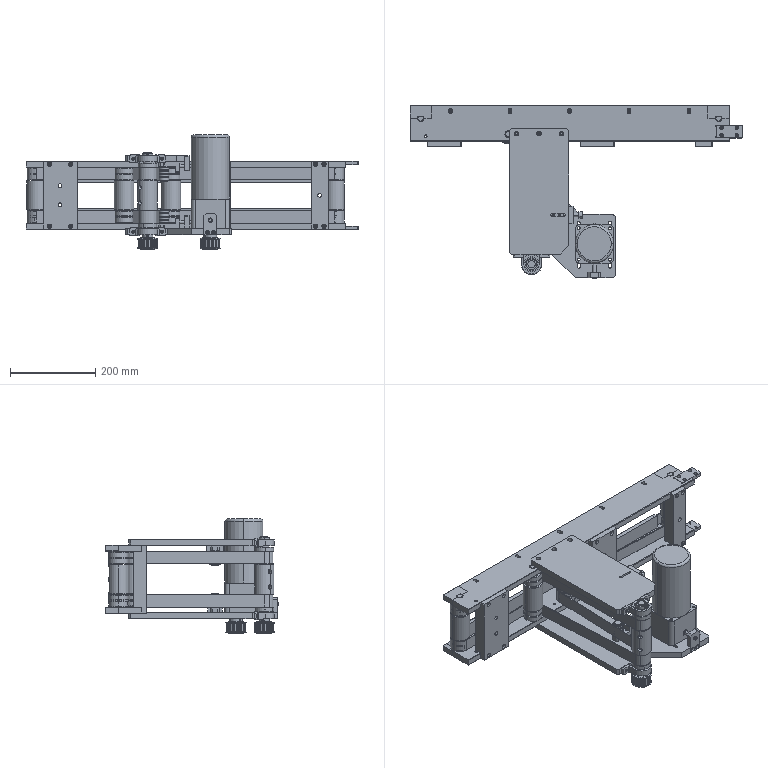Assembly | SolidWorks | mm | 105 component files | 105 solids | 2713 faces | box 780 x 408 x 268 mm | volume 7374676 mm3 | cylinder 1325 | plane 933 | cone 249 | torus 206 | commonest cylinder face diameters 15 x136 3.3 x76 1.06 x74 1.72 x73 8 x70 37.9 x64 19.7 x64 4.2 x60
Bill of materials:
ATPA15L075_A_H15-01-2 | 1 |  | Toothed pulley-like body: cylindrical hub with axial teeth/grooves around its outside, a flange at each end with an angled (chamfered) rim, and a central bore with one keyway. No extended hub.
ATPA15L075_B_H15-2 | 1 |  | Toothed pulley-like body with flanges at both ends and an extended cylindrical hub on one side. Has a central keyed bore and a radial hole through the hub.
Belt4-15^SW-111 | 1 |  | Thin-walled closed-loop band shaped like a T in plan, with a long crossbar and a tapering stem, all ends rounded; open in the middle (outline-wall only, no floor visible).
Belt5-16^SW-111 | 1 |  | Thin-walled closed-loop band shaped like a T in plan, with a long crossbar and a tapering stem, rounded ends; hollow interior.
hex head bolts-full thread grade c gb | 1 |  | Hex-head bolt-like part: hexagonal head with chamfered top corners and a round bearing face underneath, plus a plain cylindrical shank with a chamfered tip.
JBM5120-502-01-2 | 1 |  | Tall cylindrical body with a rounded top edge, sitting on a square block/flange with rounded corners and four corner through-holes; a small stepped boss and a thin round shaft stick out of the bottom face.
M8Screw-2 | 2 |  | Headed pin: a plain cylindrical shank ending in a shorter, larger-diameter cylindrical head with a flat end face.
Headless_pin_DIN_913_M4x4-2 | 4 |  | Short solid cylinder with a hexagonal socket recess in one end; both ends are chamfered, one more heavily (conical) than the other.
PBT17x-2 | 2 |  | Housing with a cylindrical body and a central through-bore, plus two side mounting ears that each have a through-hole; a round boss sticks out from one face, and the ears sit on a raised base line.
B6302ZZ-2 | 16 |  | Annular ring/disc with a central bore and rounded outer edges; the face has a raised inner rim and outer rim with a shallow recessed annulus between them.
XT-1-08-2 | 2 |  | Long slender cylindrical pin with chamfered ends and a small radial cross-hole near mid-length.
XT-1-09-2 | 24 |  | Thin flat ring (washer-like annulus) with rectangular cross-section and no visible chamfers.
XT-1-11-2 | 2 |  | Cylindrical sleeve/spacer with a coaxial through-bore and small chamfers on the outer end edges.
XT-1-07-2 | 2 |  | Long slender cylindrical pin with a small radial cross-hole near mid-length and a flat (D-cut) running along part of its length; ends chamfered.
XT-1-10-2 | 2 |  | Plain cylindrical sleeve/spacer with a concentric through bore and small chamfers on both outer end edges.
B6901ZZ-2 | 8 |  | Short thick ring with a concentric bore and a thin circular groove on the end face, between the bore and the outer edge. Slightly faceted mesh surface.
XT-1-20-2 | 2 |  | Rectangular block with a stepped, L-shaped side profile: a long thinner arm with one rounded end, and a taller square section at the other end. The arm has an elongated through opening with flat sides, a round through hole, and a cross hole in its side face.
XT-1-21-2 | 2 |  | Headed cylindrical pin: a short larger-diameter disc head on a long round shank, with a flat cut on one side of the shank near the end opposite the head.
XT-1-22-2 | 8 |  | Thin flat annular ring/washer with a large central opening and square-cut edges.
XT-1-01-2 | 1 |  | Long, narrow rectangular bar/plate with stepped notched ends, a row of oblong slots, several round holes of various sizes, small holes in the side edge, and a rectangular pocket/recess at one end.
XT-1-02-2 | 1 |  | Long, narrow rectangular bar/plate almost the same as the companion bar: stepped notched ends, a row of small slots, round holes near the middle and small side holes. The end recess looks oriented on the opposite side.
XT-1-03-2 | 2 |  | Rectangular plate with a rebated (stepped) back: a raised rectangular boss or land runs across the middle of one face. Has six through holes: four small ones near the corners and two larger ones on the centreline.
XT-1-04-2 | 1 |  | Long, slender strip with an L-shaped (angle) cross-section that has a small lip at the top. Ends have small chamfers. No holes are visible.
XT-1-05-2 | 1 |  | Long, slender strip with an L-shaped cross-section: a tall web and a short foot. A row of small, evenly spaced holes runs along its top edge.
XT-1-06-2 | 1 |  | Elongated rectangular bar or block with a stepped profile: a thinner full-length plate section carries a thicker raised section that stops short of both ends. The ends form thin flange steps. The flat face has four small through holes, one near each corner, and one larger hole in the middle.
XT-1-12-2 | 1 |  | Flat plate of even thickness with an irregular outline. A rectangular main area joins, through an angled (chamfered) edge transition, an offset rectangular extension. The extension has a large obround (slot-shaped) central cutout with four parallel elongated slots around it. The plate also has an extra slot, small holes, a rectangular notch in one edge, broken corners and small holes drilled into the edges.
XT-1-13-2 | 1 |  | Long, slender solid cylindrical shaft. One end steps down to a shorter section with a smaller diameter. Several small radial holes or dimples sit along the main length.
XT-1-14-2 | 1 |  | Stepped cylindrical sleeve with an axial bore through it. A wider band sits in the middle, with smaller-diameter ends on both sides. Three small axial holes are spaced around the end face, and the middle band has radial holes.
XT-1-15-2 | 2 |  | Round flanged disc. A smaller cylindrical boss projects from one face, a central bore runs through the part, and three holes pass through the flange.
XT-1-16-2 | 1 |  | Elongated prismatic bar or key-like block. One end is rounded into a half-round profile, and the other end looks flat or slightly angled.
XT-1-17-2 | 1 |  | Thick rectangular block. Two corners at one end are chamfered. A larger hole passes through near the chamfered end, and two smaller holes pass through near the opposite end.
XT-1-18-2 | 4 |  | Rectangular block with a semicircular U-shaped notch cut through one long edge. Two cross holes run through the block on either side of the notch, and the edges are bevelled or chamfered.
XT-1-19-2 | 1 |  | Rectangular plate or block with chamfered corners and one central through hole.
XT-1-23-2 | 1 |  | Rectangular plate or block with chamfered corners. Two smaller through holes sit near one edge, and one larger hole sits centred near the opposite edge.
XT-1-24-2 | 2 |  | Flat rectangular plate with four chamfered corners and four through holes in a rectangular pattern.
XT-1-25-2 | 1 |  | Thin, elongated rectangular plate. It has corner chamfers, one of them larger, a row of three holes along one short edge and an elongated slot near one long edge. Small holes are drilled into the side edges, and a shallow step or rebate runs along part of one edge.
Mates:
1. coincident | XT-1-01-2-1 face at (214.283, 139.385, 7.5) dir (-1, 0, 0) | XT-1-02-2-1 face at (214.283, 139.385, -138) dir (-1, 0, 0)
2. coincident | XT-1-01-2-1 face at (214.283, 54.385, 7.5) dir (0, -1, 0) | XT-1-02-2-1 face at (214.283, 54.385, -138) dir (0, -1, 0)
3. distance | XT-1-02-2-1 face at (214.283, 139.385, -138) dir (0, 0, 1) | XT-1-01-2-1 face at (214.283, 139.385, -7.5) dir (0, 0, -1)
4. coincident | XT-1-01-2-1 face at (214.283, 54.385, 7.5) dir (0, -1, 0) | XT-1-03-2-1 face at (334.283, 54.385, 7.5) dir (0, 1, 0)
5. coincident | XT-1-02-2-1 face at (214.283, 139.385, -138) dir (0, 0, 1) | XT-1-04-2-1 face at (909.283, 121.385, -138) dir (0, 0, -1)
6. distance | XT-1-04-2-1 face at (909.283, 129.385, -138) dir (0, 1, 0) | XT-1-02-2-1 face at (214.283, 139.385, -138) dir (0, 1, 0)
7. width | XT-1-04-2-1 face at (909.283, 131.385, -103) dir (1, 0, 0) | XT-1-04-2-1 face at (269.283, 131.385, -103) dir (-1, 0, 0) | XT-1-02-2-1 face at (214.283, 139.385, -138) dir (-1, 0, 0) | XT-1-02-2-1 face at (964.283, 139.385, -138) dir (1, 0, 0)
8. coincident | XT-1-01-2-1 face at (214.283, 139.385, -7.5) dir (0, 0, -1) | XT-1-05-2-1 face at (269.283, 121.385, -7.5) dir (0, 0, 1)
9. distance | XT-1-05-2-1 face at (269.283, 129.385, -7.5) dir (0, 1, 0) | XT-1-01-2-1 face at (214.283, 139.385, 7.5) dir (0, 1, 0)
10. width | XT-1-05-2-1 face at (909.283, 131.385, -42.5) dir (1, 0, 0) | XT-1-05-2-1 face at (269.283, 131.385, -42.5) dir (-1, 0, 0) | XT-1-01-2-1 face at (964.283, 139.385, 7.5) dir (1, 0, 0) | XT-1-01-2-1 face at (214.283, 139.385, 7.5) dir (-1, 0, 0)
11. coincident | XT-1-01-2-1 face at (214.283, 54.385, 7.5) dir (0, -1, 0) | XT-1-06-2-1 face at (924.283, 54.385, -138) dir (0, 1, 0)
12. concentric | XT-1-01-2-1 face at (239.283, 108.385, -7.5) dir (0, 0, 1) r 7.5 | Roller-2-1/XT-1-07-2-1 face at (239.283, 108.385, 7.5) dir (0, 0, -1) r 7.5
13. coincident | XT-1-01-2-1 face at (214.283, 139.385, 7.5) dir (0, 0, 1) | Roller-2-1/XT-1-07-2-1 face at (239.283, 108.385, 7.5) dir (0, 0, 1)
14. parallel | XT-1-01-2-1 face at (214.283, 108.385, -7.5) dir (0, 1, 0) | Roller-2-1/XT-1-07-2-1 face at (233.693, 113.385, -7.5) dir (0, 1, 0)
15. concentric | XT-1-01-2-1 face at (939.283, 108.385, -7.5) dir (0, 0, 1) r 7.5 | Roller-2-2/XT-1-07-2-1 face at (939.283, 108.385, 7.5) dir (0, 0, -1) r 7.5
16. coincident | XT-1-01-2-1 face at (214.283, 139.385, 7.5) dir (0, 0, 1) | Roller-2-2/XT-1-07-2-1 face at (939.283, 108.385, 7.5) dir (0, 0, 1)
17. parallel | XT-1-01-2-1 face at (964.283, 108.385, -7.5) dir (0, 1, 0) | Roller-2-2/XT-1-07-2-1 face at (933.693, 113.385, -7.5) dir (0, 1, 0)
18. concentric | XT-1-01-2-1 face at (444.783, 71.385, -7.5) dir (0, 0, 1) r 7.5 | Roller-01-2-1/XT-1-08-2-1 face at (444.783, 71.385, 7.5) dir (0, 0, -1) r 7.5
19. coincident | XT-1-01-2-1 face at (214.283, 139.385, 7.5) dir (0, 0, 1) | Roller-01-2-1/XT-1-08-2-1 face at (444.783, 71.385, 7.5) dir (0, 0, 1)
20. concentric | XT-1-01-2-1 face at (554.783, 71.385, -7.5) dir (0, 0, 1) r 7.5 | Roller-01-2-2/XT-1-08-2-1 face at (554.783, 71.385, 7.5) dir (0, 0, -1) r 7.5
21. coincident | XT-1-01-2-1 face at (214.283, 139.385, 7.5) dir (0, 0, 1) | Roller-01-2-2/XT-1-08-2-1 face at (554.783, 71.385, 7.5) dir (0, 0, 1)
22. coincident | XT-1-02-2-1 face at (214.283, 139.385, -153) dir (0, 0, -1) | XT-1-12-2-1 face at (447.283, 54.385, -153) dir (0, 0, 1)
23. concentric | XT-1-02-2-1 face at (464.283, 72.385, -153) dir (0, 0, -1) r 2.5 | XT-1-12-2-1 face at (464.283, 72.385, -166) dir (0, 0, -1) r 3.3
24. concentric | XT-1-02-2-1 face at (570.283, 72.385, -153) dir (0, 0, -1) r 2.5 | XT-1-12-2-1 face at (570.283, 72.385, -166) dir (0, 0, -1) r 3.3
25. coincident | XT-1-01-2-1 face at (214.283, 139.385, 7.5) dir (0, 0, 1) | XT-1-25-2-1 face at (587.283, 54.385, 7.5) dir (0, 0, -1)
26. concentric | XT-1-01-2-1 face at (570.283, 72.385, 7.5) dir (0, 0, 1) r 2.5 | XT-1-25-2-1 face at (570.283, 72.385, 20.5) dir (0, 0, 1) r 5.5
27. concentric | XT-1-01-2-1 face at (464.283, 72.385, 7.5) dir (0, 0, 1) r 2.5 | XT-1-25-2-1 face at (464.283, 72.385, 20.5) dir (0, 0, 1) r 5.5
28. coincident | XT-1-12-2-1 face at (547.283, -210.615, -151) dir (0, -1, 0) | PBT17-2-1/PBT17x-2-1 face at (457.283, -210.615, -167.5) dir (0, 1, 0)
29. concentric | XT-1-12-2-1 face at (533.283, -210.615, -158.5) dir (0, -1, 0) r 2.5 | PBT17-2-1/PBT17x-2-1 face at (533.283, -219.615, -158.5) dir (0, 1, 0) r 3.5
30. concentric | XT-1-12-2-1 face at (466.283, -210.615, -158.5) dir (0, -1, 0) r 2.5 | PBT17-2-1/PBT17x-2-1 face at (466.283, -219.615, -158.5) dir (0, 1, 0) r 3.5
31. coincident | XT-1-25-2-1 face at (447.283, -210.615, 20.5) dir (0, -1, 0) | PBT17-2-2/PBT17x-2-1 face at (542.283, -210.615, 22) dir (0, 1, 0)
32. concentric | XT-1-25-2-1 face at (466.283, -210.615, 13) dir (0, -1, 0) r 2.5 | PBT17-2-2/PBT17x-2-1 face at (466.283, -219.615, 13) dir (0, 1, 0) r 3.5
33. concentric | XT-1-25-2-1 face at (533.283, -210.615, 13) dir (0, -1, 0) r 2.5 | PBT17-2-2/PBT17x-2-1 face at (533.283, -219.615, 13) dir (0, 1, 0) r 3.5
34. concentric | PBT17-2-1/PBT17x-2-1 face at (499.783, -234.615, -153.5) dir (0, 0, -1) r 8.5 | XT-1-13-2-1 face at (499.783, -234.615, -199) dir (0, 0, -1) r 8.5
35. distance | XT-1-13-2-1 face at (499.783, -234.615, 28.5) dir (0, 0, 1) | PBT17-2-2/PBT17x-2-1 face at (499.783, -246.865, 25.5) dir (0, 0, 1)
36. concentric | XT-1-13-2-1 face at (499.783, -234.615, -199) dir (0, 0, -1) r 8.5 | XT-1-14-2-1 face at (499.783, -234.615, -138.5) dir (0, 0, 1) r 8.5
37. concentric | XT-1-13-2-1 face at (492.915, -239.623, -90.75) dir (-0.8081, -0.5891, 0) r 2.6 | XT-1-14-2-1 face at (481.602, -247.87, -90.75) dir (-0.8081, -0.5891, 0) r 2.75
38. concentric | XT-1-13-2-1 face at (499.783, -234.615, -199) dir (0, 0, -1) r 8.5 | XT-1-15-2-1 face at (499.783, -234.615, -138.5) dir (0, 0, -1) r 8.5
39. concentric | XT-1-14-2-1 face at (484.868, -236.208, -138.5) dir (0, 0, -1) r 1.65 | XT-1-15-2-1 face at (484.868, -236.208, -148.5) dir (0, 0, -1) r 4
40. coincident | XT-1-14-2-1 face at (488.001, -218.454, -138.5) dir (0, 0, -1) | XT-1-15-2-1 face at (499.783, -234.615, -138.5) dir (0, 0, 1)
41. concentric | XT-1-13-2-1 face at (499.783, -234.615, -199) dir (0, 0, -1) r 8.5 | XT-1-15-2-2 face at (499.783, -234.615, -7) dir (0, 0, 1) r 8.5
42. concentric | XT-1-14-2-1 face at (493.705, -248.328, -7) dir (0, 0, 1) r 1.65 | XT-1-15-2-2 face at (493.705, -248.328, 3) dir (0, 0, 1) r 4
43. coincident | XT-1-14-2-1 face at (499.783, -234.615, -7) dir (0, 0, 1) | XT-1-15-2-2 face at (499.783, -234.615, -7) dir (0, 0, -1)
44. coincident | XT-1-12-2-1 face at (447.283, 84.385, -151) dir (0, 0, 1) | JBM5120-502-01-2-1 face at (692.283, -231.615, -151) dir (0, 0, -1)
45. width | XT-1-12-2-1 face at (680.533, -136.615, -151) dir (1, 0, 0) | XT-1-12-2-1 face at (687.533, -136.615, -151) dir (-1, 0, 0) | JBM5120-502-01-2-1 face at (684.033, -149.865, 69) dir (0, 0, -1) r 3.5
46. width | XT-1-12-2-1 face at (607.033, -136.615, -151) dir (1, 0, 0) | XT-1-12-2-1 face at (614.033, -136.615, -151) dir (-1, 0, 0) | JBM5120-502-01-2-1 face at (610.533, -149.865, 69) dir (0, 0, -1) r 3.5
47. distance | JBM5120-502-01-2-1 face at (692.283, -141.615, -81.5) dir (0, 1, 0) | XT-1-12-2-1 face at (697.283, -116.615, -166) dir (0, 1, 0)
48. concentric | XT-1-13-2-1 face at (499.783, -234.615, -199) dir (0, 0, -1) r 7.5 | ATPA15L075_A_H15-01-2-1 face at (499.783, -234.615, -211) dir (0, 0, 1) r 7.5
49. coincident | XT-1-13-2-1 face at (504.202, -240.676, -199) dir (0, 0, -1) | ATPA15L075_A_H15-01-2-1 face at (494.776, -227.747, -199) dir (0, 0, -1)
50. coincident | XT-1-13-2-1 face at (497.132, -230.979, -199) dir (-0.5891, 0.8081, 0) | XT-1-16-2-1 face at (497.132, -230.979, -175) dir (0.5891, -0.8081, 0)
51. coincident | XT-1-13-2-1 face at (495.516, -232.157, -199) dir (0.8081, 0.5891, 0) | XT-1-16-2-1 face at (492.571, -228.117, -175) dir (-0.8081, -0.5891, 0)
52. coincident | XT-1-13-2-1 face at (504.202, -240.676, -199) dir (0, 0, -1) | XT-1-16-2-1 face at (495.803, -225.76, -199) dir (0, 0, -1)
53. coincident | ATPA15L075_A_H15-01-2-1 face at (492.142, -227.528, -173) dir (0.8081, 0.5891, 0) | XT-1-16-2-1 face at (492.571, -228.117, -175) dir (-0.8081, -0.5891, 0)
54. concentric | JBM5120-502-01-2-1 face at (647.283, -168.115, -189.5) dir (0, 0, 1) r 7.5 | ATPA15L075_B_H15-2-1 face at (647.283, -168.115, -161) dir (0, 0, -1) r 7.5
55. coincident | ATPA15L075_A_H15-01-2-1 face at (494.776, -227.747, -199) dir (0, 0, -1) | ATPA15L075_B_H15-2-1 face at (657.801, -181.851, -199) dir (0, 0, -1)
56. coincident | XT-1-12-2-1 face at (662.283, -253.615, -151) dir (0, -1, 0) | XT-1-17-2-1 face at (632.333, -253.615, -166) dir (0, 1, 0)
57. concentric | XT-1-12-2-1 face at (640.283, -253.615, -160) dir (0, -1, 0) r 2.1 | XT-1-17-2-1 face at (640.283, -265.615, -160) dir (0, -1, 0) r 5
58. concentric | XT-1-12-2-1 face at (654.283, -253.615, -160) dir (0, -1, 0) r 2.1 | XT-1-17-2-1 face at (654.283, -265.615, -160) dir (0, -1, 0) r 5
59. concentric | XT-1-17-2-1 face at (647.283, -253.615, -131) dir (0, 1, 0) r 5 | hex head bolts-full thread grade c gb-1 face at (647.283, -268.615, -131) dir (0, 1, 0) r 4
60. distance | hex head bolts-full thread grade c gb-1 face at (647.283, -268.615, -131) dir (0, -1, 0) | XT-1-17-2-1 face at (632.333, -265.615, -166) dir (0, -1, 0)
61. concentric | XT-1-02-2-1 face at (923.783, 108.385, -145.5) dir (0, 1, 0) r 2.1 | XT-1-18-2-1 face at (923.783, 139.385, -145.5) dir (0, 1, 0) r 5
62. concentric | XT-1-02-2-1 face at (954.783, 108.385, -145.5) dir (0, 1, 0) r 2.1 | XT-1-18-2-1 face at (954.783, 139.385, -145.5) dir (0, 1, 0) r 5
63. coincident | XT-1-02-2-1 face at (964.283, 108.385, -153) dir (0, 1, 0) | XT-1-18-2-1 face at (964.283, 108.385, -153) dir (0, -1, 0)
64. coincident | XT-1-02-2-1 face at (214.283, 108.385, -153) dir (0, 1, 0) | XT-1-18-2-2 face at (231.783, 108.385, -153) dir (0, -1, 0)
65. concentric | XT-1-02-2-1 face at (254.783, 108.385, -145.5) dir (0, 1, 0) r 2.1 | XT-1-18-2-2 face at (254.783, 139.385, -145.5) dir (0, 1, 0) r 5
66. concentric | XT-1-02-2-1 face at (223.783, 108.385, -145.5) dir (0, 1, 0) r 2.1 | XT-1-18-2-2 face at (223.783, 139.385, -145.5) dir (0, 1, 0) r 2.75
67. concentric | XT-1-01-2-1 face at (254.783, 108.385, 0) dir (0, 1, 0) r 2.1 | XT-1-18-2-3 face at (254.783, 139.385, 0) dir (0, 1, 0) r 2.75
68. concentric | XT-1-01-2-1 face at (223.783, 108.385, 0) dir (0, 1, 0) r 2.1 | XT-1-18-2-3 face at (223.783, 139.385, 0) dir (0, 1, 0) r 2.75
69. coincident | XT-1-01-2-1 face at (214.283, 108.385, -7.5) dir (0, 1, 0) | XT-1-18-2-3 face at (214.283, 108.385, 7.5) dir (0, -1, 0)
70. concentric | XT-1-01-2-1 face at (954.783, 108.385, 0) dir (0, 1, 0) r 2.1 | XT-1-18-2-4 face at (954.783, 139.385, 0) dir (0, 1, 0) r 2.75
71. concentric | XT-1-01-2-1 face at (923.783, 108.385, 0) dir (0, 1, 0) r 2.1 | XT-1-18-2-4 face at (923.783, 139.385, 0) dir (0, 1, 0) r 2.75
72. coincident | XT-1-01-2-1 face at (964.283, 108.385, -7.5) dir (0, 1, 0) | XT-1-18-2-4 face at (946.783, 108.385, 7.5) dir (0, -1, 0)
73. lock to sketch | assembly sketch segment at (264.283, 139.385, -7.5) dir (1, 0, 0) | assembly sketch segment at (264.283, 139.385, -7.5) dir (0, 1, 0) | Belt4-15^SW-111-1 sketch segment at (264.283, 139.385, -7.5) dir (1, 0, 0) | Belt4-15^SW-111-1 sketch segment at (264.283, 139.385, -7.5) dir (0, 1, 0)
74. lock to sketch | assembly sketch segment at (214.283, 139.385, -138) dir (1, 0, 0) | assembly sketch segment at (214.283, 139.385, -138) dir (0, 1, 0) | Belt5-16^SW-111-1 sketch segment at (214.283, 139.385, -138) dir (1, 0, 0) | Belt5-16^SW-111-1 sketch segment at (214.283, 139.385, -138) dir (0, 1, 0)
75. coincident | XT-1-01-2-1 face at (214.283, 54.385, 7.5) dir (0, -1, 0) | XT-1-03-2-2 face at (694.283, 54.385, 7.5) dir (0, 1, 0)
76. concentric | XT-1-01-2-1 face at (894.283, 54.385, 0) dir (0, -1, 0) r 2.1 | XT-1-06-2-1 face at (894.283, 42.385, 0) dir (0, -1, 0) r 2.75
77. concentric | XT-1-01-2-1 face at (914.283, 54.385, 0) dir (0, -1, 0) r 2.1 | XT-1-06-2-1 face at (914.283, 42.385, 0) dir (0, -1, 0) r 2.75
78. concentric | XT-1-01-2-1 face at (679.283, 54.385, 0) dir (0, -1, 0) r 2.1 | XT-1-03-2-2 face at (679.283, 42.385, 0) dir (0, -1, 0) r 2.75
79. concentric | XT-1-01-2-1 face at (629.283, 54.385, 0) dir (0, -1, 0) r 2.1 | XT-1-03-2-2 face at (629.283, 42.385, 0) dir (0, -1, 0) r 2.75
80. concentric | XT-1-01-2-1 face at (319.283, 54.385, 0) dir (0, -1, 0) r 2.1 | XT-1-03-2-1 face at (319.283, 42.385, 0) dir (0, -1, 0) r 2.75
81. concentric | XT-1-01-2-1 face at (269.283, 54.385, 0) dir (0, -1, 0) r 2.1 | XT-1-03-2-1 face at (269.283, 42.385, 0) dir (0, -1, 0) r 2.75
82. coincident | XT-1-12-2-1 face at (447.283, 84.385, -151) dir (0, 0, 1) | TensioningWheel-2-1/XT-1-20-2-1 face at (526.036, -108.615, -151) dir (0, 0, -1)
83. width | XT-1-12-2-1 face at (577.283, -115.965, -151) dir (0, -1, 0) | XT-1-12-2-1 face at (577.283, -121.265, -151) dir (0, 1, 0) | TensioningWheel-2-1/XT-1-20-2-1 face at (551.036, -118.615, -151) dir (0, 0, -1) r 2.1
84. width | XT-1-12-2-1 face at (577.283, -115.965, -151) dir (0, -1, 0) | XT-1-12-2-1 face at (577.283, -121.265, -151) dir (0, 1, 0) | TensioningWheel-2-1/XT-1-20-2-1 face at (566.036, -118.615, -151) dir (0, 0, -1) r 2.1
85. coincident | XT-1-25-2-1 face at (447.283, 84.385, 5.5) dir (0, 0, -1) | TensioningWheel-2-2/XT-1-20-2-1 face at (526.036, -128.615, 5.5) dir (0, 0, 1)
86. coincident | TensioningWheel-2-1/XT-1-20-2-1 face at (526.036, -108.615, -140) dir (0, 1, 0) | TensioningWheel-2-2/XT-1-20-2-1 face at (526.036, -108.615, -5.5) dir (0, 1, 0)
87. coincident | TensioningWheel-2-1/XT-1-20-2-1 face at (576.036, -108.615, -140) dir (1, 0, 0) | TensioningWheel-2-2/XT-1-20-2-1 face at (576.036, -128.615, -5.5) dir (1, 0, 0)
88. coincident | XT-1-25-2-1 face at (587.283, -265.615, 5.5) dir (1, 0, 0) | XT-1-23-2-1 face at (587.283, -98.615, 20.5) dir (-1, 0, 0)
89. coincident | XT-1-25-2-1 face at (447.283, 84.385, 20.5) dir (0, 0, 1) | XT-1-23-2-1 face at (597.283, -98.615, 20.5) dir (0, 0, 1)
90. width | XT-1-23-2-1 face at (597.283, -98.615, 20.5) dir (0, 1, 0) | XT-1-23-2-1 face at (597.283, -138.615, 20.5) dir (0, -1, 0) | TensioningWheel-2-2/XT-1-20-2-1 face at (526.036, -108.615, -5.5) dir (0, 1, 0) | TensioningWheel-2-2/XT-1-20-2-1 face at (526.036, -128.615, -5.5) dir (0, -1, 0)
91. concentric | XT-1-23-2-1 face at (597.283, -118.615, -4.5) dir (1, 0, 0) r 4 | M8Screw-2-1 face at (619.036, -118.615, -4.5) dir (1, 0, 0) r 4
92. coincident | TensioningWheel-2-2/XT-1-20-2-1 face at (576.036, -128.615, -5.5) dir (1, 0, 0) | M8Screw-2-1 face at (576.036, -118.615, -4.5) dir (-1, 0, 0)
93. coincident | XT-1-12-2-1 face at (447.283, 84.385, -151) dir (0, 0, 1) | XT-1-19-2-1 face at (587.283, -101.115, -151) dir (0, 0, -1)
94. coincident | XT-1-23-2-1 face at (597.283, -98.615, 20.5) dir (1, 0, 0) | XT-1-19-2-1 face at (597.283, -101.115, -151) dir (1, 0, 0)
95. width | XT-1-19-2-1 face at (587.283, -101.115, -151) dir (0, 1, 0) | XT-1-19-2-1 face at (587.283, -136.115, -151) dir (0, -1, 0) | TensioningWheel-2-1/XT-1-20-2-1 face at (526.036, -108.615, -140) dir (0, 1, 0) | TensioningWheel-2-1/XT-1-20-2-1 face at (526.036, -128.615, -140) dir (0, -1, 0)
96. concentric | XT-1-19-2-1 face at (587.283, -118.615, -136) dir (-1, 0, 0) r 4 | M8Screw-2-2 face at (619.036, -118.615, -136) dir (1, 0, 0) r 4
97. coincident | M8Screw-2-1 face at (619.036, -115.363, -11.809) dir (1, 0, 0) | M8Screw-2-2 face at (619.036, -115.363, -143.309) dir (1, 0, 0)
98. coincident | XT-1-02-2-1 face at (214.283, 139.385, -145) dir (0, 0, -1) | XT-1-24-2-2 face at (994.283, 62.385, -145) dir (0, 0, 1)
99. concentric | XT-1-02-2-1 face at (946.283, 86.385, -145) dir (0, 0, -1) r 1.65 | XT-1-24-2-2 face at (946.283, 86.385, -153) dir (0, 0, -1) r 2.15
100. concentric | XT-1-02-2-1 face at (946.283, 68.385, -145) dir (0, 0, -1) r 1.65 | XT-1-24-2-2 face at (946.283, 68.385, -153) dir (0, 0, -1) r 2.15
101. coincident | XT-1-01-2-1 face at (214.283, 139.385, -0.5) dir (0, 0, 1) | XT-1-24-2-5 face at (934.283, 62.385, -0.5) dir (0, 0, -1)
102. concentric | XT-1-01-2-1 face at (946.283, 86.385, -0.5) dir (0, 0, 1) r 1.65 | XT-1-24-2-5 face at (946.283, 86.385, 7.5) dir (0, 0, 1) r 2.15
103. concentric | XT-1-01-2-1 face at (946.283, 68.385, -0.5) dir (0, 0, 1) r 1.65 | XT-1-24-2-5 face at (946.283, 68.385, 7.5) dir (0, 0, 1) r 2.15
104. tangent | Belt5-16^SW-111-1 face at (534.783, 96.348, -109) dir (0.9992, -0.0407, 0) | TensioningWheel-2-1/B6901ZZ-2-3 face at (538.036, -118.615, -124) dir (0, 0, -1) r 12
105. distance | Headless_pin_DIN_913_M4x4-2-1 plane at (0, 32.5, 9.406) dir (0, -1, 0) | PBT17x-2-1 plane at (0, 32.5, 0) dir (0, 1, 0)
106. coincident | PBT17x-2-1 axis at (0, 50, 9.406) dir (0, -1, 0) | Headless_pin_DIN_913_M4x4-2-1 axis at (0, -44.4, 9.406) dir (0, 1, 0)
107. coincident | PBT17x-2-1 axis at (0, 50, 9.406) dir (0, -1, 0) | Headless_pin_DIN_913_M4x4-2-1 axis at (0, -44.4, 9.406) dir (0, 1, 0)
108. coincident | PBT17x-2-1 axis at (0, 50, 9.406) dir (0, -1, 0) | Headless_pin_DIN_913_M4x4-2-1 axis at (0, -44.4, 9.406) dir (0, 1, 0)
109. angle | Headless_pin_DIN_913_M4x4-2-1 plane at (0, 36.5, 9.406) dir (1, 0, 0) | PBT17x-2-1 plane at (0, 0, 0) dir (1, 0, 0)
110. distance | Headless_pin_DIN_913_M4x4-2-2 plane at (-7.361, 19.75, 9.406) dir (0.866, 0.5, 0) | PBT17x-2-1 plane at (3.031, 1.75, 0) dir (-0.866, -0.5, 0)
111. coincident | PBT17x-2-1 axis at (-80.454, -22.45, 9.406) dir (0.866, 0.5, 0) | Headless_pin_DIN_913_M4x4-2-2 axis at (59.236, 58.2, 9.406) dir (-0.866, -0.5, 0)
112. coincident | PBT17x-2-1 axis at (-80.454, -22.45, 9.406) dir (0.866, 0.5, 0) | Headless_pin_DIN_913_M4x4-2-2 axis at (59.236, 58.2, 9.406) dir (-0.866, -0.5, 0)
113. coincident | PBT17x-2-1 axis at (-80.454, -22.45, 9.406) dir (0.866, 0.5, 0) | Headless_pin_DIN_913_M4x4-2-2 axis at (59.236, 58.2, 9.406) dir (-0.866, -0.5, 0)
114. angle | Headless_pin_DIN_913_M4x4-2-2 plane at (-10.825, 17.75, 9.406) dir (0.5, -0.866, 0) | PBT17x-2-1 plane at (-10.392, 18, 0) dir (0.5, -0.866, 0)
115. concentric | XT-1-08-2-1 face at (0.2889, 1.187, 160.5) dir (0, 0, -1) r 7.5 | XT-1-11-2-1 face at (0.2889, 1.187, 115) dir (0, 0, -1) r 7.5
116. concentric | XT-1-08-2-1 face at (0.2889, 9.687, 80.25) dir (0, 1, 0) r 1.65 | XT-1-11-2-1 face at (0.2889, 24.187, 80.25) dir (0, 1, 0) r 4
117. concentric | XT-1-08-2-1 face at (0.2889, 1.187, 160.5) dir (0, 0, -1) r 7.5 | XT-1-09-2-1 face at (0.2889, 1.187, 116.5) dir (0, 0, -1) r 7.5
118. coincident | XT-1-11-2-1 face at (0.2889, 1.187, 115) dir (0, 0, 1) | XT-1-09-2-1 face at (0.2889, 1.187, 115) dir (0, 0, -1)
119. concentric | XT-1-08-2-1 face at (0.2889, 1.187, 160.5) dir (0, 0, -1) r 7.5 | XT-1-09-2-2 face at (0.2889, 1.187, 45.5) dir (0, 0, -1) r 7.5
120. coincident | XT-1-11-2-1 face at (0.2889, 1.187, 45.5) dir (0, 0, -1) | XT-1-09-2-2 face at (0.2889, 1.187, 45.5) dir (0, 0, 1)
121. concentric | XT-1-08-2-1 face at (0.2889, 1.187, 160.5) dir (0, 0, -1) r 7.5 | XT-1-09-2-3 face at (0.2889, 1.187, 31) dir (0, 0, -1) r 7.5
122. concentric | XT-1-08-2-1 face at (0.2889, 1.187, 160.5) dir (0, 0, -1) r 7.5 | XT-1-09-2-4 face at (0.2889, 1.187, 16.5) dir (0, 0, -1) r 7.5
123. concentric | XT-1-08-2-1 face at (0.2889, 1.187, 160.5) dir (0, 0, -1) r 7.5 | XT-1-09-2-5 face at (0.2889, 1.187, 131) dir (0, 0, -1) r 7.5
124. concentric | XT-1-08-2-1 face at (0.2889, 1.187, 160.5) dir (0, 0, -1) r 7.5 | XT-1-09-2-6 face at (0.2889, 1.187, 145.5) dir (0, 0, -1) r 7.5
125. concentric | XT-1-08-2-1 face at (0.2889, 1.187, 160.5) dir (0, 0, -1) r 7.5 | B6302ZZ-2-1 face at (0.2889, 1.187, 116.5) dir (0, 0, 1) r 7.5
126. coincident | XT-1-09-2-1 face at (0.2889, 1.187, 116.5) dir (0, 0, 1) | B6302ZZ-2-1 face at (0.2889, 9.687, 116.5) dir (0, 0, -1)
127. concentric | XT-1-08-2-1 face at (0.2889, 1.187, 160.5) dir (0, 0, -1) r 7.5 | B6302ZZ-2-2 face at (0.2889, 1.187, 131) dir (0, 0, 1) r 7.5
128. coincident | XT-1-09-2-5 face at (0.2889, 1.187, 131) dir (0, 0, 1) | B6302ZZ-2-2 face at (0.2205, 9.686, 131) dir (0, 0, -1)
129. concentric | XT-1-08-2-1 face at (0.2889, 1.187, 160.5) dir (0, 0, -1) r 7.5 | B6302ZZ-2-3 face at (0.2889, 1.187, 31) dir (0, 0, 1) r 7.5
130. coincident | XT-1-09-2-2 face at (0.2889, 1.187, 44) dir (0, 0, -1) | B6302ZZ-2-3 face at (0.2096, 11.036, 44) dir (0, 0, 1)
131. coincident | XT-1-09-2-3 face at (0.2889, 1.187, 31) dir (0, 0, 1) | B6302ZZ-2-3 face at (0.2205, 9.686, 31) dir (0, 0, -1)
132. coincident | XT-1-09-2-6 face at (0.2889, 1.187, 144) dir (0, 0, -1) | B6302ZZ-2-2 face at (0.2096, 11.036, 144) dir (0, 0, 1)
133. concentric | XT-1-08-2-1 face at (0.2889, 1.187, 160.5) dir (0, 0, -1) r 7.5 | B6302ZZ-2-4 face at (0.2889, 1.187, 16.5) dir (0, 0, 1) r 7.5
134. coincident | XT-1-09-2-3 face at (0.2889, 1.187, 29.5) dir (0, 0, -1) | B6302ZZ-2-4 face at (0.2096, 11.036, 29.5) dir (0, 0, 1)
135. coincident | XT-1-09-2-4 face at (0.2889, 1.187, 16.5) dir (0, 0, 1) | B6302ZZ-2-4 face at (0.2205, 9.686, 16.5) dir (0, 0, -1)
136. concentric | XT-1-07-2-1 face at (4.437, 0.9597, 160.5) dir (0, 0, -1) r 7.5 | XT-1-10-2-1 face at (4.437, 0.9597, 115) dir (0, 0, -1) r 7.5
137. concentric | XT-1-07-2-1 face at (12.937, 0.9597, 80.25) dir (1, 0, 0) r 1.65 | XT-1-10-2-1 face at (27.437, 0.9597, 80.25) dir (1, 0, 0) r 2.25
138. concentric | XT-1-07-2-1 face at (4.437, 0.9597, 160.5) dir (0, 0, -1) r 7.5 | XT-1-09-2-1 face at (4.437, 0.9597, 116.5) dir (0, 0, -1) r 7.5
139. coincident | XT-1-10-2-1 face at (4.437, 0.9597, 115) dir (0, 0, 1) | XT-1-09-2-1 face at (4.437, 0.9597, 115) dir (0, 0, -1)
140. concentric | XT-1-07-2-1 face at (4.437, 0.9597, 160.5) dir (0, 0, -1) r 7.5 | XT-1-09-2-2 face at (4.437, 0.9597, 131) dir (0, 0, -1) r 7.5
141. concentric | XT-1-07-2-1 face at (4.437, 0.9597, 160.5) dir (0, 0, -1) r 7.5 | XT-1-09-2-3 face at (4.437, 0.9597, 145.5) dir (0, 0, -1) r 7.5
142. concentric | XT-1-07-2-1 face at (4.437, 0.9597, 160.5) dir (0, 0, -1) r 7.5 | XT-1-09-2-4 face at (4.437, 0.9597, 45.5) dir (0, 0, -1) r 7.5
143. coincident | XT-1-10-2-1 face at (4.437, 0.9597, 45.5) dir (0, 0, -1) | XT-1-09-2-4 face at (4.437, 0.9597, 45.5) dir (0, 0, 1)
144. concentric | XT-1-07-2-1 face at (4.437, 0.9597, 160.5) dir (0, 0, -1) r 7.5 | XT-1-09-2-5 face at (4.437, 0.9597, 31) dir (0, 0, -1) r 7.5
145. concentric | XT-1-07-2-1 face at (4.437, 0.9597, 160.5) dir (0, 0, -1) r 7.5 | XT-1-09-2-6 face at (4.437, 0.9597, 16.5) dir (0, 0, -1) r 7.5
146. concentric | XT-1-07-2-1 face at (4.437, 0.9597, 160.5) dir (0, 0, -1) r 7.5 | B6302ZZ-2-1 face at (4.437, 0.9597, 116.5) dir (0, 0, 1) r 7.5
147. coincident | XT-1-09-2-1 face at (4.437, 0.9597, 116.5) dir (0, 0, 1) | B6302ZZ-2-1 face at (4.437, 9.46, 116.5) dir (0, 0, -1)
148. coincident | XT-1-09-2-2 face at (4.437, 0.9597, 129.5) dir (0, 0, -1) | B6302ZZ-2-1 face at (4.437, 10.81, 129.5) dir (0, 0, 1)
149. concentric | XT-1-07-2-1 face at (4.437, 0.9597, 160.5) dir (0, 0, -1) r 7.5 | B6302ZZ-2-2 face at (4.437, 0.9597, 131) dir (0, 0, 1) r 7.5
150. coincident | XT-1-09-2-2 face at (4.437, 0.9597, 131) dir (0, 0, 1) | B6302ZZ-2-2 face at (4.437, 9.46, 131) dir (0, 0, -1)
151. coincident | XT-1-09-2-3 face at (4.437, 0.9597, 144) dir (0, 0, -1) | B6302ZZ-2-2 face at (4.437, 10.81, 144) dir (0, 0, 1)
152. concentric | XT-1-07-2-1 face at (4.437, 0.9597, 160.5) dir (0, 0, -1) r 7.5 | B6302ZZ-2-3 face at (4.437, 0.9597, 31) dir (0, 0, 1) r 7.5
153. coincident | XT-1-09-2-4 face at (4.437, 0.9597, 44) dir (0, 0, -1) | B6302ZZ-2-3 face at (4.437, 10.81, 44) dir (0, 0, 1)
154. coincident | XT-1-09-2-5 face at (4.437, 0.9597, 31) dir (0, 0, 1) | B6302ZZ-2-3 face at (4.437, 9.46, 31) dir (0, 0, -1)
155. concentric | XT-1-07-2-1 face at (4.437, 0.9597, 160.5) dir (0, 0, -1) r 7.5 | B6302ZZ-2-4 face at (4.437, 0.9597, 16.5) dir (0, 0, 1) r 7.5
156. coincident | XT-1-09-2-5 face at (4.437, 0.9597, 29.5) dir (0, 0, -1) | B6302ZZ-2-4 face at (6.695, 10.548, 29.5) dir (0, 0, 1)
157. coincident | XT-1-09-2-6 face at (4.437, 0.9597, 16.5) dir (0, 0, 1) | B6302ZZ-2-4 face at (6.385, 9.233, 16.5) dir (0, 0, -1)
158. concentric | XT-1-20-2-1 face at (-6.085, 1.433, 5.5) dir (0, 0, -1) r 6 | XT-1-21-2-1 face at (-6.085, 1.433, 40.5) dir (0, 0, 1) r 6
159. coincident | XT-1-20-2-1 face at (-18.085, 11.433, -5.5) dir (0, 0, -1) | XT-1-21-2-1 face at (-6.085, 1.433, -5.5) dir (0, 0, -1)
160. coincident | XT-1-20-2-1 face at (-10.557, 5.433, 5.5) dir (0, -1, 0) | XT-1-21-2-1 face at (-10.557, 5.433, 5.5) dir (0, 1, 0)
161. concentric | XT-1-21-2-1 face at (-6.085, 1.433, 40.5) dir (0, 0, 1) r 6 | B6901ZZ-2-1 face at (-6.085, 1.433, 37.5) dir (0, 0, -1) r 6
162. coincident | XT-1-21-2-1 face at (-0.08529, 1.433, 37.5) dir (0, 0, -1) | B6901ZZ-2-1 face at (-6.085, 7.733, 37.5) dir (0, 0, 1)
163. concentric | XT-1-21-2-1 face at (-6.085, 1.433, 40.5) dir (0, 0, 1) r 6 | XT-1-22-2-1 face at (-6.085, 1.433, 31.5) dir (0, 0, -1) r 6.05
164. coincident | B6901ZZ-2-1 face at (-6.085, 9.233, 31.5) dir (0, 0, -1) | XT-1-22-2-1 face at (-6.085, 1.433, 31.5) dir (0, 0, 1)
165. concentric | XT-1-21-2-1 face at (-6.085, 1.433, 40.5) dir (0, 0, 1) r 6 | B6901ZZ-2-2 face at (-6.085, 1.433, 29.5) dir (0, 0, -1) r 6
166. coincident | XT-1-22-2-1 face at (-6.085, 1.433, 29.5) dir (0, 0, -1) | B6901ZZ-2-2 face at (-6.085, 7.733, 29.5) dir (0, 0, 1)
167. concentric | XT-1-22-2-1 face at (-6.085, 1.433, 31.5) dir (0, 0, -1) r 8 | XT-1-22-2-2 face at (-6.085, 1.433, 23.5) dir (0, 0, -1) r 6.05
168. coincident | B6901ZZ-2-2 face at (-6.085, 9.233, 23.5) dir (0, 0, -1) | XT-1-22-2-2 face at (-6.085, 1.433, 23.5) dir (0, 0, 1)
169. concentric | XT-1-21-2-1 face at (-6.085, 1.433, 40.5) dir (0, 0, 1) r 6 | B6901ZZ-2-3 face at (-6.085, 1.433, 21.5) dir (0, 0, -1) r 6
170. coincident | B6901ZZ-2-3 face at (-6.085, 7.733, 21.5) dir (0, 0, 1) | XT-1-22-2-2 face at (-6.085, 1.433, 21.5) dir (0, 0, -1)
171. concentric | XT-1-21-2-1 face at (-6.085, 1.433, 40.5) dir (0, 0, 1) r 6 | XT-1-22-2-3 face at (-6.085, 1.433, 15.5) dir (0, 0, -1) r 6.05
172. coincident | B6901ZZ-2-3 face at (-6.085, 9.233, 15.5) dir (0, 0, -1) | XT-1-22-2-3 face at (-6.085, 1.433, 15.5) dir (0, 0, 1)
173. concentric | XT-1-21-2-1 face at (-6.085, 1.433, 40.5) dir (0, 0, 1) r 6 | B6901ZZ-2-4 face at (-6.085, 1.433, 13.5) dir (0, 0, -1) r 6
174. coincident | XT-1-22-2-3 face at (-6.085, 1.433, 13.5) dir (0, 0, -1) | B6901ZZ-2-4 face at (-6.25, 7.731, 13.5) dir (0, 0, 1)
175. coincident | B6901ZZ-2-4 face at (-6.289, 9.23, 7.5) dir (0, 0, -1) | XT-1-22-2-4 face at (-6.085, 1.433, 7.5) dir (0, 0, 1)
176. concentric | XT-1-21-2-1 face at (-6.085, 1.433, 40.5) dir (0, 0, 1) r 6 | XT-1-22-2-4 face at (-6.085, 1.433, 7.5) dir (0, 0, -1) r 6.05